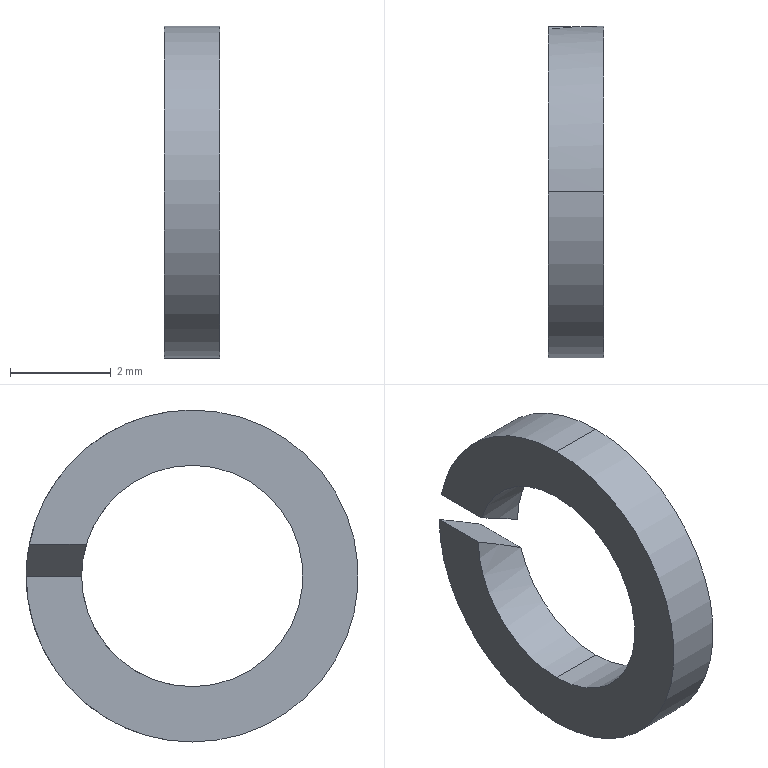Component | SolidWorks | spring lock washers--normal type gb-1 | 1 solid | 10 faces | box 1.1 x 6.6 x 6.6 mm | volume 20 mm3 | cylinder 6 | plane 4 | commonest cylinder face diameters 4.4 x3 6.6 x3
build123d program:
from build123d import *

# Parameters (mm, degrees)
SKETCH1_R          = 3.3
SKETCH1_R_2        = 2.2
BASE_EXTRUDE_DEPTH = 1.1
CUT_EXTRUDE1_DEPTH = 5.795


with BuildPart() as part:
    # Sketch1 → Base-Extrude (new body)
    with BuildSketch(Plane.XY):
        Circle(SKETCH1_R)
        Circle(SKETCH1_R_2, mode=Mode.SUBTRACT)
    extrude(amount=-BASE_EXTRUDE_DEPTH)

    # Sketch2 → Cut-Extrude1 (cut, through all)
    with BuildSketch(Plane(origin=(0, 0, 0), x_dir=(1, 0, 0), z_dir=(0, 1, 0))):
        Polygon((0, 1.1), (0.6351, 0), (0, 0), (-0.6351, 1.1), align=None)
    extrude(amount=CUT_EXTRUDE1_DEPTH, mode=Mode.SUBTRACT)


solid = part.part

# Placed as in the assembly
solid = solid.moved(Location((149.337, -33.063, -275.554), (0, 90, 0)))